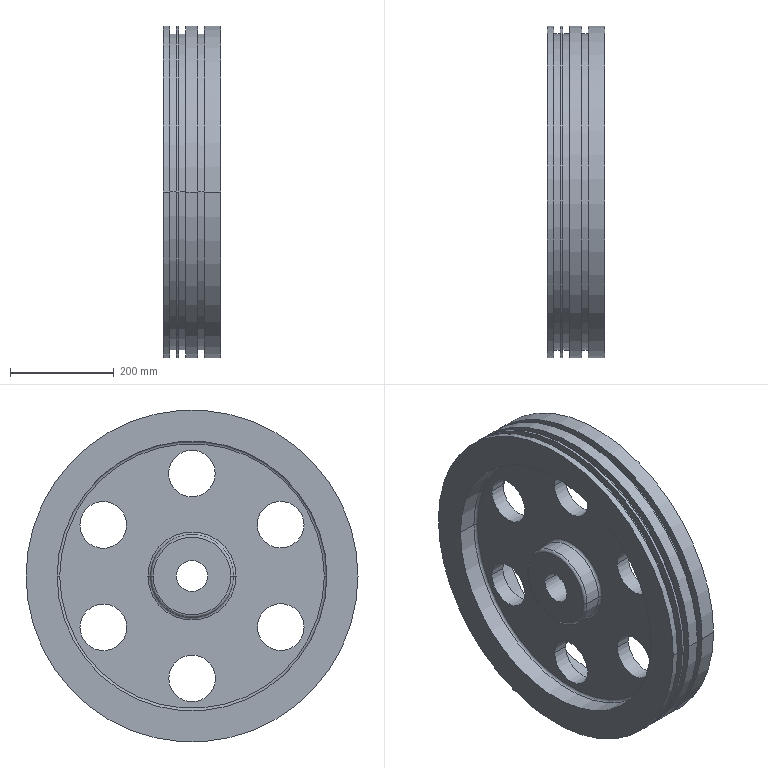Component | SolidWorks | LargePulley-1 | 1 solid | 53 faces | box 110 x 640 x 640 mm | volume 16754461 mm3 | cylinder 34 | plane 11 | torus 8 | commonest cylinder face diameters 90 x12 640 x8 610 x6 520 x4 60 x2 160 x2
build123d program:
from build123d import *

# Parameters (mm, degrees)
SKETCH1_2_W                                     = 320
SKETCH1_2_H                                     = 110
HOLE1_D                                         = 520
HOLE1_DEPTH                                     = 41.574
SKETCH4_W                                       = 80
SKETCH4_H                                       = 41.574
M56_HEX_HEAD_BOLT_COUNTERBORE_HOLE1_D           = 60
M56_HEX_HEAD_BOLT_COUNTERBORE_HOLE1_CBORE_D     = 520
M56_HEX_HEAD_BOLT_COUNTERBORE_HOLE1_CBORE_DEPTH = 38.426
M80_CLEARANCE_HOLE1_D                           = 90
M80_CLEARANCE_HOLE1_DEPTH                       = 71.574
FILLET1_R                                       = 5
SKETCH1_R                                       = 321
SKETCH1_R_2                                     = 305
REPAIR_BELTGROOVE1_DEPTH                        = 6.5
SKETCH2_R                                       = 321
SKETCH2_R_2                                     = 305
REPAIR_BELTGROOVE2_DEPTH                        = 6.5
SKETCH3_R                                       = 321
SKETCH3_R_2                                     = 305
REPAIR_BELTGROOVE3_DEPTH                        = 6.5


with BuildPart() as part:
    # Sketch1_2 → Revolve1 (revolve)
    with BuildSketch(Plane.XZ.offset(99.787), mode=Mode.PRIVATE) as revolve1_sk:
        with Locations((617.238, 55)):
            Rectangle(SKETCH1_2_W, SKETCH1_2_H)
    revolve(revolve1_sk.sketch.rotate(Axis((457.238, -99.787, 110), (0, 0, -1)), 180), axis=Axis((457.238, -99.787, 110), (0, 0, -1)))

    # Hole1
    with Locations(Plane(origin=(0, 0, 0), x_dir=(-1, 0, 0), z_dir=(0, 0, -1))):
        with Locations((-457.238, -99.787)):
            Hole(HOLE1_D / 2, depth=HOLE1_DEPTH)

    # Sketch4 → Revolve2 (revolve)
    with BuildSketch(Plane(origin=(0, -99.787, 0), x_dir=(1, 0, 0), z_dir=(0, 1, 0)), mode=Mode.PRIVATE) as revolve2_sk:
        with Locations((497.238, -20.787)):
            Rectangle(SKETCH4_W, SKETCH4_H)
    revolve(revolve2_sk.sketch.rotate(Axis((457.238, -99.787, 0), (0, 0, 1)), 180), axis=Axis((457.238, -99.787, 0), (0, 0, 1)))

    # M56 Hex Head Bolt Counterbore Hole1 (through all)
    with Locations(Plane.XY.offset(110)):
        with Locations((457.238, -99.787)):
            CounterBoreHole(M56_HEX_HEAD_BOLT_COUNTERBORE_HOLE1_D / 2, M56_HEX_HEAD_BOLT_COUNTERBORE_HOLE1_CBORE_D / 2, M56_HEX_HEAD_BOLT_COUNTERBORE_HOLE1_CBORE_DEPTH)

    # M80 Clearance Hole1
    with Locations(Plane.XY.offset(71.574)):
        with Locations((286.078, -198.328), (457.479, 97.713), (456.997, -297.287), (628.158, -198.745), (286.319, -0.8282), (628.398, -1.246)):
            Hole(M80_CLEARANCE_HOLE1_D / 2, depth=M80_CLEARANCE_HOLE1_DEPTH)

    # Fillet1
    fillet1_edges = [part.edges().sort_by_distance(p)[0] for p in [
        (197.238, -99.787, 41.574),
        (537.238, -99.787, 0),
        (537.238, -99.787, 41.574),
        (197.238, -99.787, 71.574),
    ]]
    fillet(fillet1_edges, radius=FILLET1_R)

    # Sketch1 → Repair_BeltGroove1 (cut, symmetric)
    with BuildSketch(Plane.XY.offset(18.32)):
        with Locations((457.238, -99.787)):
            Circle(SKETCH1_R)
        with Locations((457.238, -99.787)):
            Circle(SKETCH1_R_2, mode=Mode.SUBTRACT)
    extrude(amount=REPAIR_BELTGROOVE1_DEPTH, both=True, mode=Mode.SUBTRACT)

    # Sketch2 → Repair_BeltGroove2 (cut, symmetric)
    with BuildSketch(Plane.XY.offset(36.32)):
        with Locations((457.238, -99.787)):
            Circle(SKETCH2_R)
        with Locations((457.238, -99.787)):
            Circle(SKETCH2_R_2, mode=Mode.SUBTRACT)
    extrude(amount=REPAIR_BELTGROOVE2_DEPTH, both=True, mode=Mode.SUBTRACT)

    # Sketch3 → Repair_BeltGroove3 (cut, symmetric)
    with BuildSketch(Plane.XY.offset(72.32)):
        with Locations((457.238, -99.787)):
            Circle(SKETCH3_R)
        with Locations((457.238, -99.787)):
            Circle(SKETCH3_R_2, mode=Mode.SUBTRACT)
    extrude(amount=REPAIR_BELTGROOVE3_DEPTH, both=True, mode=Mode.SUBTRACT)


solid = part.part

# Placed as in the assembly
solid = solid.moved(Location((-903.339, 878.528, 1114.384), (90, 90, 0)))